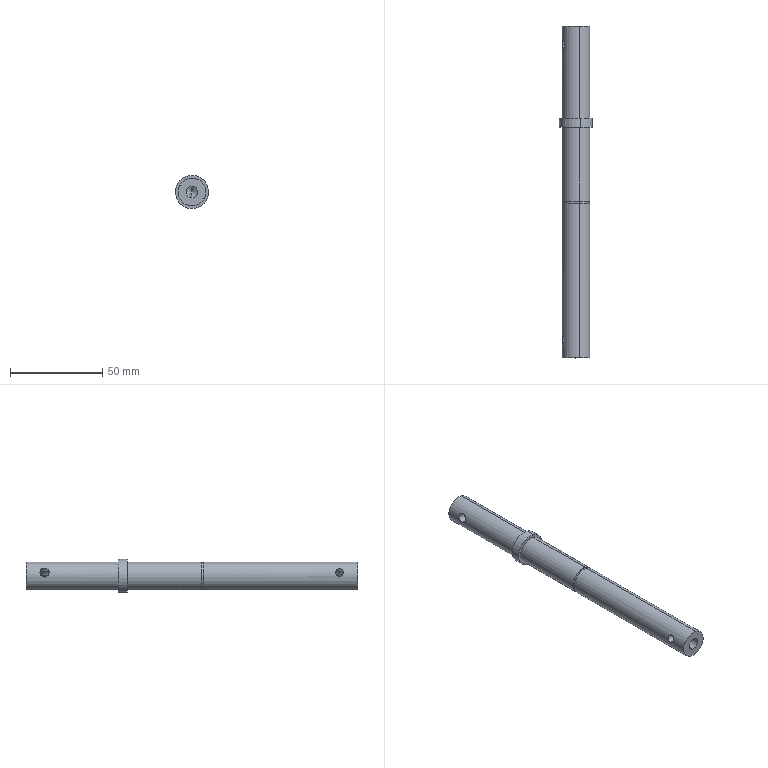Component | SolidWorks | 75-02-21StirringRod-1 | 1 solid | 31 faces | box 18 x 180 x 18 mm | volume 30040 mm3 | cylinder 22 | plane 7 | cone 2 | commonest cylinder face diameters 15 x6 4.2 x4 5 x4 6.4 x2 14.3 x2 6 x2 18 x2 | material A3 Steel
build123d program:
from build123d import *

# Parameters (mm, degrees)
F_6_4_6_4_DIAMETER_HOLE1_D     = 6.4
F_6_4_6_4_DIAMETER_HOLE1_DEPTH = 30
F_6_4_6_4_DIAMETER_HOLE1_TIP   = 1.923
M5_TAPPED_HOLE1_D              = 4.2
SKETCH8_R                      = 3
CUT_EXTRUDE1_DEPTH             = 30
M6_TAPPED_HOLE1_D              = 5
SKETCH12_R                     = 7.5
SKETCH12_R_2                   = 7.15
CUT_EXTRUDE2_DEPTH             = 1.1


with BuildPart() as part:
    # Sketch1 → Revolve1 (revolve)
    with BuildSketch(Plane.XY, mode=Mode.PRIVATE) as revolve1_sk:
        Polygon((0, 0), (0, 7.5), (125, 7.5), (125, 9), (130, 9), (130, 7.5), (180, 7.5), (180, 0), align=None)
    revolve(revolve1_sk.sketch.rotate(Axis((-32.122, 0, 0), (1, 0, 0)), 90), axis=Axis((-32.122, 0, 0), (1, 0, 0)))

    # 6.4 _6.4_ Diameter Hole1
    with Locations(Plane(origin=(0, 0, 0), x_dir=(0, 0, -1), z_dir=(-1, 0, 0))):
        with Locations((0, 0)):
            Hole(F_6_4_6_4_DIAMETER_HOLE1_D / 2, depth=F_6_4_6_4_DIAMETER_HOLE1_DEPTH)
            with Locations((0, 0, -(F_6_4_6_4_DIAMETER_HOLE1_DEPTH + F_6_4_6_4_DIAMETER_HOLE1_TIP / 2))):  # 118° drill point
                Cone(0, F_6_4_6_4_DIAMETER_HOLE1_D / 2, F_6_4_6_4_DIAMETER_HOLE1_TIP, mode=Mode.SUBTRACT)

    # M5 Tapped Hole1 (through all)
    with Locations(Plane(origin=(0, 10, 0), x_dir=(1, 0, 0), z_dir=(0, 1, 0))):
        with Locations((10, 0)):
            Hole(M5_TAPPED_HOLE1_D / 2)

    # Sketch8 → Cut-Extrude1 (cut)
    with BuildSketch(Plane(origin=(180, 0, 0), x_dir=(0, 0, -1), z_dir=(1, 0, 0))):
        Circle(SKETCH8_R)
    extrude(amount=-CUT_EXTRUDE1_DEPTH, mode=Mode.SUBTRACT)

    # M6 Tapped Hole1 (through all)
    with Locations(Plane(origin=(170, 7.5, 0), x_dir=(0, 0, 1), z_dir=(0, 1, 0))):
        with Locations((0, 0)):
            Hole(M6_TAPPED_HOLE1_D / 2)

    # Sketch12 → Cut-Extrude2 (cut)
    with BuildSketch(Plane.ZY.offset(-85)):
        Circle(SKETCH12_R)
        Circle(SKETCH12_R_2, mode=Mode.SUBTRACT)
    extrude(amount=CUT_EXTRUDE2_DEPTH, mode=Mode.SUBTRACT)


solid = part.part

# Placed as in the assembly
solid = solid.moved(Location((-17.87, 110.856, -43.68), (180, -15.261, -90)))